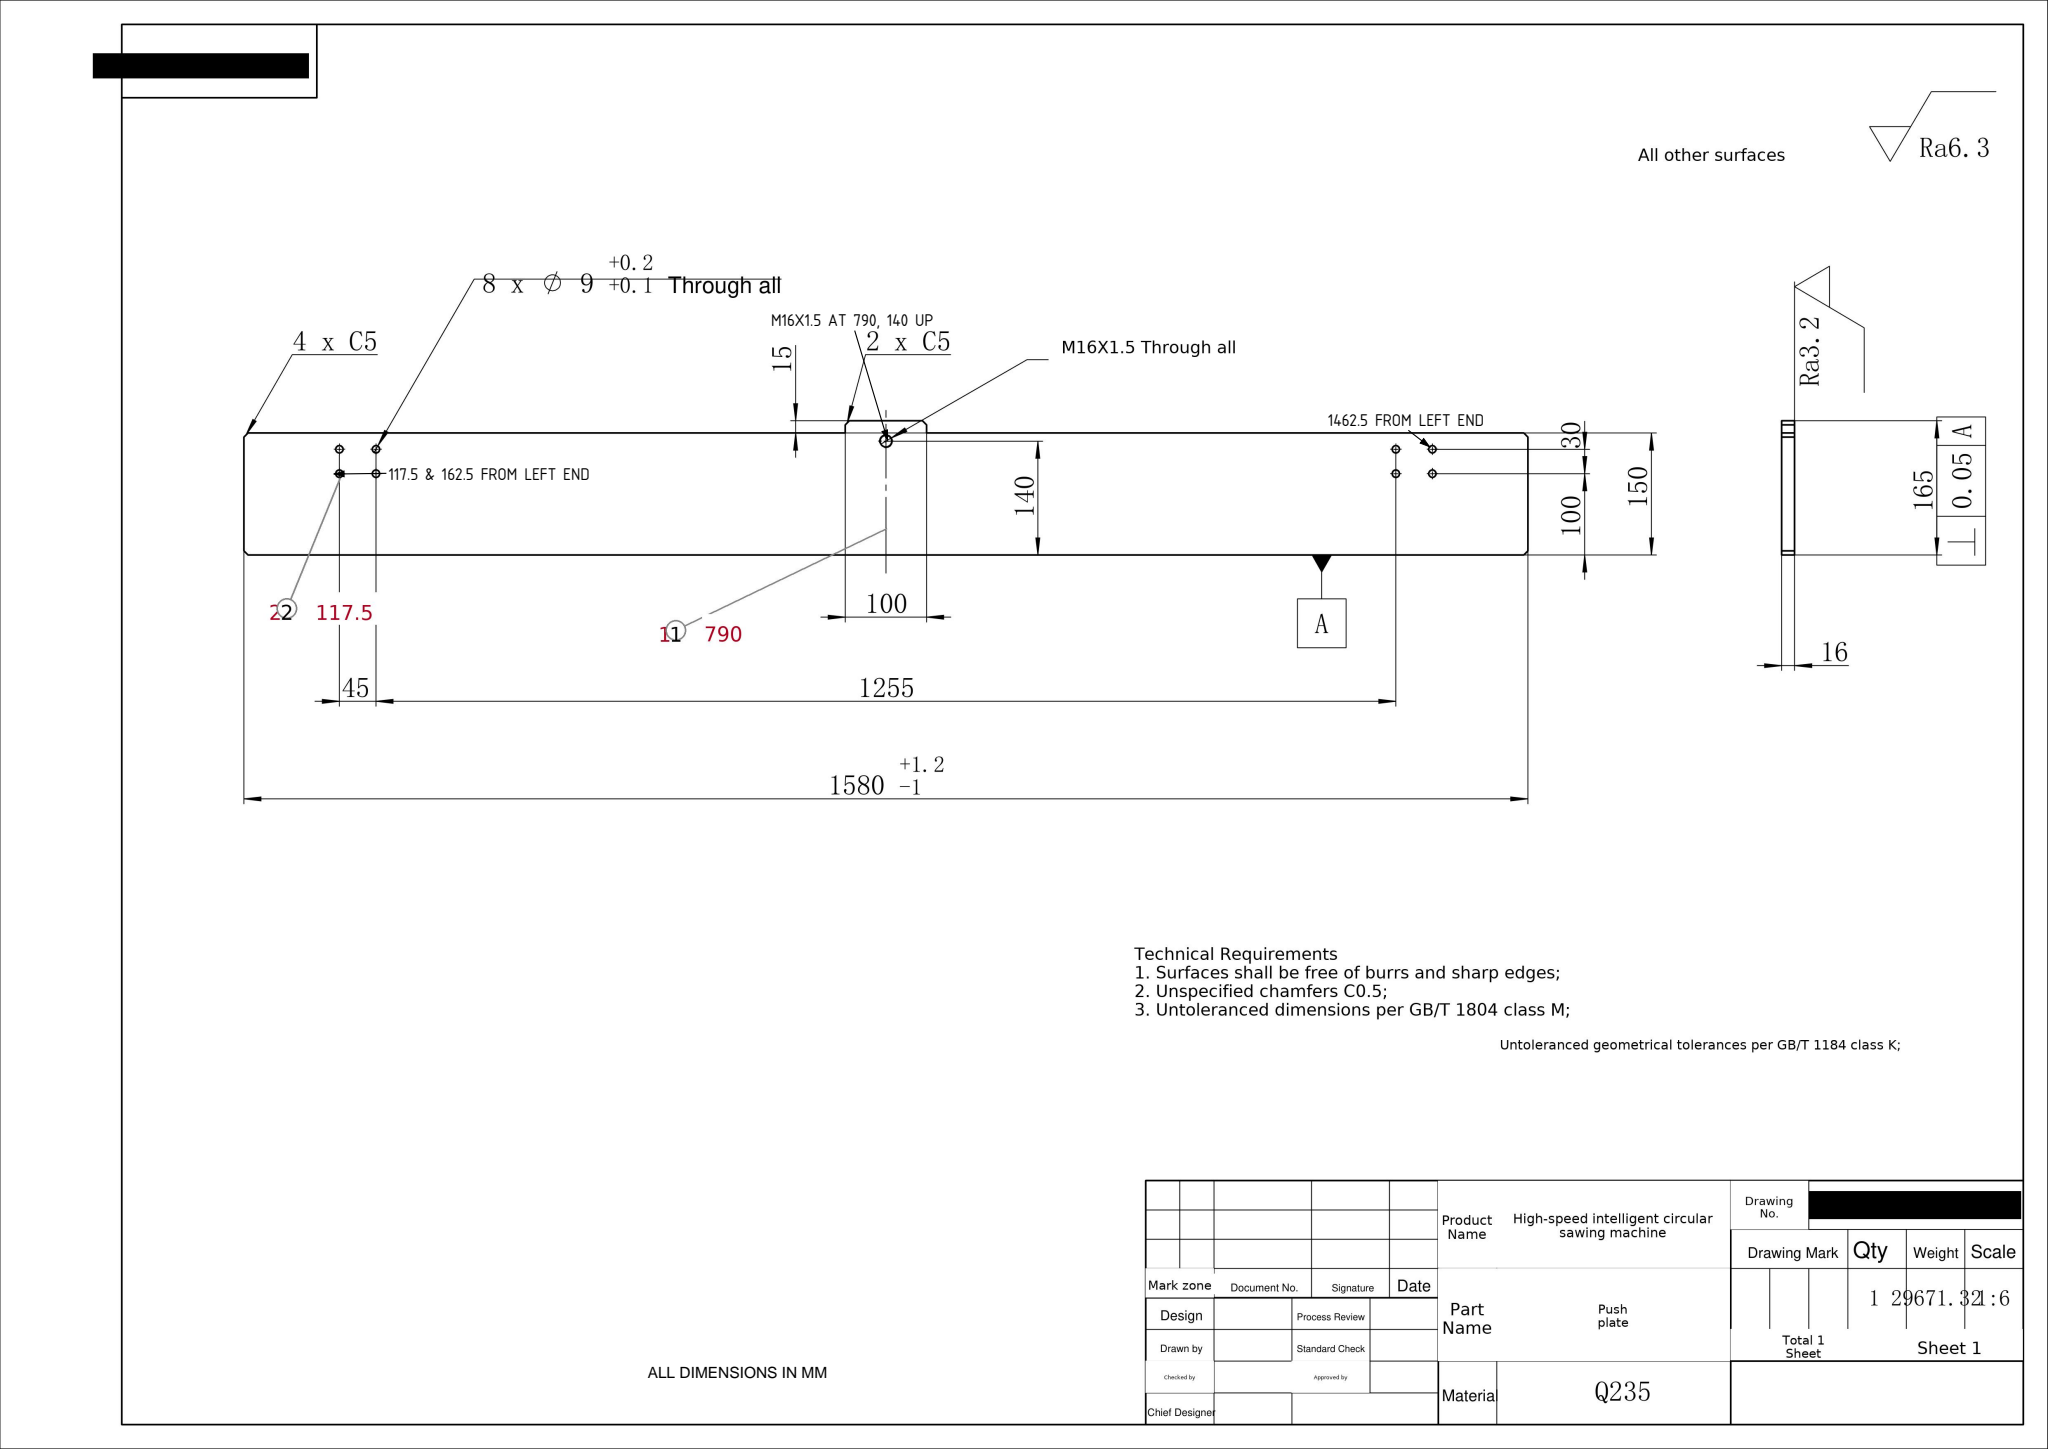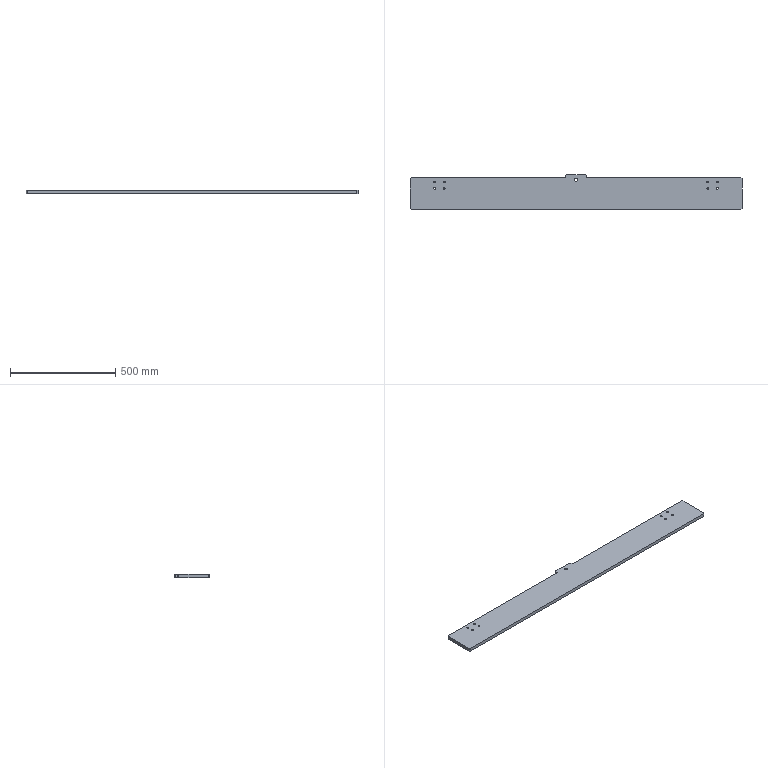Part | SolidWorks | mm | material Q235 | 1 solid | 34 faces | box 1580 x 165 x 16 mm | volume 3804015 mm3 | cylinder 18 | plane 16 | commonest cylinder face diameters 9 x16 14.5 x2
Drawing notes:
RH Ø9 OUTER HOLE COL: 1462.5 FROM LH END | from the solid: Ø9 cylinders at x=1462.5 (y=100 & 130), bbox x length 1580
Ø9 HOLE COL 117.5 FROM LEFT END; NEXT COL 162.5 | from the solid: Ø9 z-axis holes at x=117.5 and x=162.5 (also 1417.5/1462.5), L=16 thru
M16X1.5 THRU 790 FROM LEFT END, 140 FROM BOTTOM EDGE | from the solid: Ø14.5 z-axis hole at x=790.0, y=140.0, length 16 (bbox 1580x165x16)
build123d program:
from build123d import *

# Parameters (mm, degrees)
SKETCH1_W                = 1580
SKETCH1_H                = 150
BOSS_EXTRUDE1_DEPTH      = 16
F_9_0_9_DIAMETER_HOLE1_D = 9
SKETCH4_W                = 100
SKETCH4_H                = 15
BOSS_EXTRUDE2_DEPTH      = 16
M16X1_5_TAPPED_HOLE1_D   = 14.5
CHAMFER1_SIZE            = 5


with BuildPart() as part:
    # Sketch1 → Boss-Extrude1 (new body)
    with BuildSketch(Plane.XY):
        with Locations((790, 75)):
            Rectangle(SKETCH1_W, SKETCH1_H)
    extrude(amount=BOSS_EXTRUDE1_DEPTH)

    # 9.0 _9_ Diameter Hole1 (through all)
    with Locations(Plane.XY.offset(16)):
        with Locations((117.5, 130), (162.5, 130), (117.5, 100), (162.5, 100), (1417.5, 100), (1462.5, 100), (1417.5, 130), (1462.5, 130)):
            Hole(F_9_0_9_DIAMETER_HOLE1_D / 2)

    # Sketch4 → Boss-Extrude2 (add)
    with BuildSketch(Plane.XY.offset(16)):
        with Locations((790, 157.5)):
            Rectangle(SKETCH4_W, SKETCH4_H)
    extrude(amount=-BOSS_EXTRUDE2_DEPTH)

    # M16x1.5 Tapped Hole1 (through all)
    with Locations(Plane.XY.offset(16)):
        with Locations((790, 140)):
            Hole(M16X1_5_TAPPED_HOLE1_D / 2)

    # Chamfer1
    chamfer1_edges = [part.edges().sort_by_distance(p)[0] for p in [
        (740, 165, 8),
        (840, 165, 8),
        (0, 150, 8),
        (1580, 150, 8),
        (1580, 0, 8),
        (0, 0, 8),
    ]]
    chamfer(chamfer1_edges, length=CHAMFER1_SIZE)


solid = part.part